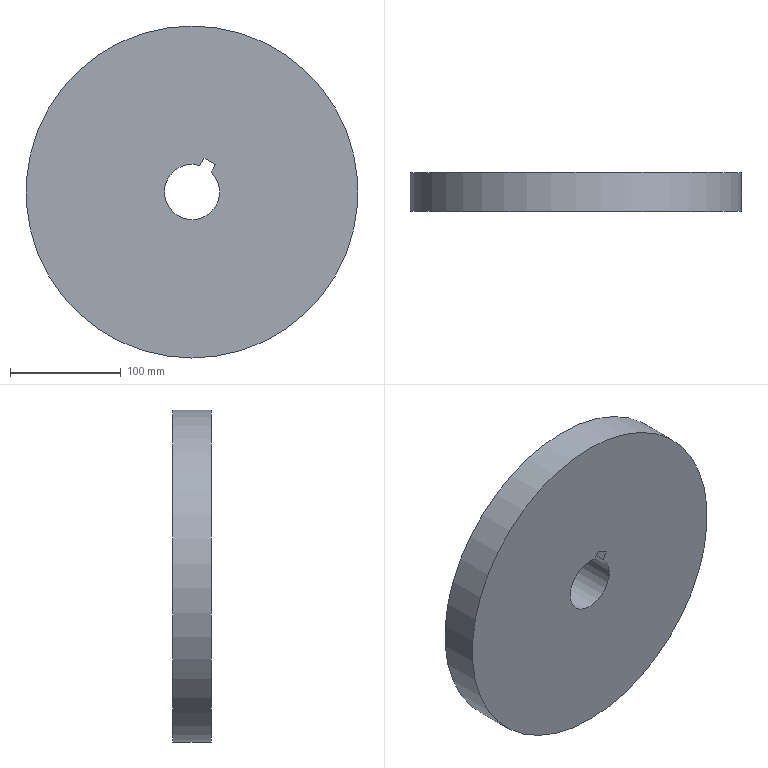Component | NX | TAS | 1 solid | 7 faces | box 300 x 35 x 300 mm | volume 2402240 mm3 | plane 5 | cylinder 2 | commonest cylinder face diameters 300 x1 50 x1
STEP:
#1=CARTESIAN_POINT('',(0.,0.,0.));
#2=DIRECTION('',(0.,0.,1.));
#3=DIRECTION('',(1.,0.,0.));
#4=AXIS2_PLACEMENT_3D('',#1,#2,#3);
#5=CARTESIAN_POINT('',(-1145.062,827.425,250.713));
#6=VERTEX_POINT('',#5);
#7=CARTESIAN_POINT('',(-1148.928,827.425,244.018));
#8=VERTEX_POINT('',#7);
#9=CARTESIAN_POINT('',(-1145.062,827.425,250.713));
#10=DIRECTION('',(-0.5,0.,-0.866));
#11=VECTOR('',#10,1.);
#12=LINE('',#9,#11);
#13=CARTESIAN_POINT('',(-1145.062,792.425,250.713));
#14=DIRECTION('',(0.866,0.,-0.5));
#15=DIRECTION('',(0.5,0.,0.866));
#16=AXIS2_PLACEMENT_3D('',#13,#14,#15);
#17=PLANE('',#16);
#18=CARTESIAN_POINT('',(0.,-35.));
#19=DIRECTION('',(-1.,0.));
#20=VECTOR('',#19,1.);
#21=LINE('',#18,#20);
#22=(GEOMETRIC_REPRESENTATION_CONTEXT(2)PARAMETRIC_REPRESENTATION_CONTEXT()REPRESENTATION_CONTEXT('',''));
#23=DEFINITIONAL_REPRESENTATION('',(#21),#22);
#24=PCURVE('',#17,#23);
#25=CARTESIAN_POINT('',(-1155.866,827.425,220.));
#26=DIRECTION('',(0.,-1.,0.));
#27=DIRECTION('',(-0.5,0.,-0.866));
#28=AXIS2_PLACEMENT_3D('',#25,#26,#27);
#29=PLANE('',#28);
#30=CARTESIAN_POINT('',(-32.,-6.));
#31=DIRECTION('',(1.,-0.));
#32=VECTOR('',#31,1.);
#33=LINE('',#30,#32);
#34=(GEOMETRIC_REPRESENTATION_CONTEXT(2)PARAMETRIC_REPRESENTATION_CONTEXT()REPRESENTATION_CONTEXT('',''));
#35=DEFINITIONAL_REPRESENTATION('',(#33),#34);
#36=PCURVE('',#29,#35);
#37=SURFACE_CURVE('',#12,(#24,#36),.PCURVE_S1.);
#38=EDGE_CURVE('',#6,#8,#37,.T.);
#39=ORIENTED_EDGE('',*,*,#38,.F.);
#40=CARTESIAN_POINT('',(-1145.062,792.425,250.713));
#41=VERTEX_POINT('',#40);
#42=CARTESIAN_POINT('',(-1145.062,792.425,250.713));
#43=DIRECTION('',(0.,1.,0.));
#44=VECTOR('',#43,1.);
#45=LINE('',#42,#44);
#46=CARTESIAN_POINT('',(0.,0.));
#47=DIRECTION('',(0.,-1.));
#48=VECTOR('',#47,1.);
#49=LINE('',#46,#48);
#50=(GEOMETRIC_REPRESENTATION_CONTEXT(2)PARAMETRIC_REPRESENTATION_CONTEXT()REPRESENTATION_CONTEXT('',''));
#51=DEFINITIONAL_REPRESENTATION('',(#49),#50);
#52=PCURVE('',#17,#51);
#53=CARTESIAN_POINT('',(-1134.67,792.425,244.713));
#54=DIRECTION('',(-0.5,0.,-0.866));
#55=DIRECTION('',(0.866,0.,-0.5));
#56=AXIS2_PLACEMENT_3D('',#53,#54,#55);
#57=PLANE('',#56);
#58=CARTESIAN_POINT('',(-12.,0.));
#59=DIRECTION('',(0.,-1.));
#60=VECTOR('',#59,1.);
#61=LINE('',#58,#60);
#62=(GEOMETRIC_REPRESENTATION_CONTEXT(2)PARAMETRIC_REPRESENTATION_CONTEXT()REPRESENTATION_CONTEXT('',''));
#63=DEFINITIONAL_REPRESENTATION('',(#61),#62);
#64=PCURVE('',#57,#63);
#65=SURFACE_CURVE('',#45,(#52,#64),.PCURVE_S1.);
#66=EDGE_CURVE('',#41,#6,#65,.T.);
#67=ORIENTED_EDGE('',*,*,#66,.F.);
#68=CARTESIAN_POINT('',(-1148.928,792.425,244.018));
#69=VERTEX_POINT('',#68);
#70=CARTESIAN_POINT('',(-1145.062,792.425,250.713));
#71=DIRECTION('',(-0.5,0.,-0.866));
#72=VECTOR('',#71,1.);
#73=LINE('',#70,#72);
#74=CARTESIAN_POINT('',(0.,0.));
#75=DIRECTION('',(-1.,0.));
#76=VECTOR('',#75,1.);
#77=LINE('',#74,#76);
#78=(GEOMETRIC_REPRESENTATION_CONTEXT(2)PARAMETRIC_REPRESENTATION_CONTEXT()REPRESENTATION_CONTEXT('',''));
#79=DEFINITIONAL_REPRESENTATION('',(#77),#78);
#80=PCURVE('',#17,#79);
#81=CARTESIAN_POINT('',(-1155.866,792.425,220.));
#82=DIRECTION('',(0.,-1.,0.));
#83=DIRECTION('',(-0.5,0.,-0.866));
#84=AXIS2_PLACEMENT_3D('',#81,#82,#83);
#85=PLANE('',#84);
#86=CARTESIAN_POINT('',(-32.,-6.));
#87=DIRECTION('',(1.,-0.));
#88=VECTOR('',#87,1.);
#89=LINE('',#86,#88);
#90=(GEOMETRIC_REPRESENTATION_CONTEXT(2)PARAMETRIC_REPRESENTATION_CONTEXT()REPRESENTATION_CONTEXT('',''));
#91=DEFINITIONAL_REPRESENTATION('',(#89),#90);
#92=PCURVE('',#85,#91);
#93=SURFACE_CURVE('',#73,(#80,#92),.PCURVE_S1.);
#94=EDGE_CURVE('',#41,#69,#93,.T.);
#95=ORIENTED_EDGE('',*,*,#94,.T.);
#96=CARTESIAN_POINT('',(-1148.928,792.425,244.018));
#97=DIRECTION('',(0.,1.,0.));
#98=VECTOR('',#97,1.);
#99=LINE('',#96,#98);
#100=CARTESIAN_POINT('',(-7.731,0.));
#101=DIRECTION('',(0.,-1.));
#102=VECTOR('',#101,1.);
#103=LINE('',#100,#102);
#104=(GEOMETRIC_REPRESENTATION_CONTEXT(2)PARAMETRIC_REPRESENTATION_CONTEXT()REPRESENTATION_CONTEXT('',''));
#105=DEFINITIONAL_REPRESENTATION('',(#103),#104);
#106=PCURVE('',#17,#105);
#107=CARTESIAN_POINT('',(-1155.866,792.425,220.));
#108=DIRECTION('',(0.,1.,0.));
#109=DIRECTION('',(0.5,0.,0.866));
#110=AXIS2_PLACEMENT_3D('',#107,#108,#109);
#111=CYLINDRICAL_SURFACE('',#110,25.);
#112=CARTESIAN_POINT('',(6.041,0.));
#113=DIRECTION('',(0.,1.));
#114=VECTOR('',#113,1.);
#115=LINE('',#112,#114);
#116=(GEOMETRIC_REPRESENTATION_CONTEXT(2)PARAMETRIC_REPRESENTATION_CONTEXT()REPRESENTATION_CONTEXT('',''));
#117=DEFINITIONAL_REPRESENTATION('',(#115),#116);
#118=PCURVE('',#111,#117);
#119=SURFACE_CURVE('',#99,(#106,#118),.PCURVE_S1.);
#120=EDGE_CURVE('',#69,#8,#119,.T.);
#121=ORIENTED_EDGE('',*,*,#120,.T.);
#122=EDGE_LOOP('',(#39,#67,#95,#121));
#123=FACE_BOUND('',#122,.T.);
#124=ADVANCED_FACE('',(#123),#17,.T.);
#125=CARTESIAN_POINT('',(-1134.67,827.425,244.713));
#126=VERTEX_POINT('',#125);
#127=CARTESIAN_POINT('',(-1134.67,827.425,244.713));
#128=DIRECTION('',(-0.866,0.,0.5));
#129=VECTOR('',#128,1.);
#130=LINE('',#127,#129);
#131=CARTESIAN_POINT('',(0.,-35.));
#132=DIRECTION('',(-1.,0.));
#133=VECTOR('',#132,1.);
#134=LINE('',#131,#133);
#135=(GEOMETRIC_REPRESENTATION_CONTEXT(2)PARAMETRIC_REPRESENTATION_CONTEXT()REPRESENTATION_CONTEXT('',''));
#136=DEFINITIONAL_REPRESENTATION('',(#134),#135);
#137=PCURVE('',#57,#136);
#138=CARTESIAN_POINT('',(-32.,6.));
#139=DIRECTION('',(-0.,-1.));
#140=VECTOR('',#139,1.);
#141=LINE('',#138,#140);
#142=(GEOMETRIC_REPRESENTATION_CONTEXT(2)PARAMETRIC_REPRESENTATION_CONTEXT()REPRESENTATION_CONTEXT('',''));
#143=DEFINITIONAL_REPRESENTATION('',(#141),#142);
#144=PCURVE('',#29,#143);
#145=SURFACE_CURVE('',#130,(#137,#144),.PCURVE_S1.);
#146=EDGE_CURVE('',#126,#6,#145,.T.);
#147=ORIENTED_EDGE('',*,*,#146,.F.);
#148=CARTESIAN_POINT('',(-1134.67,792.425,244.713));
#149=VERTEX_POINT('',#148);
#150=CARTESIAN_POINT('',(-1134.67,792.425,244.713));
#151=DIRECTION('',(0.,1.,0.));
#152=VECTOR('',#151,1.);
#153=LINE('',#150,#152);
#154=CARTESIAN_POINT('',(0.,0.));
#155=DIRECTION('',(0.,-1.));
#156=VECTOR('',#155,1.);
#157=LINE('',#154,#156);
#158=(GEOMETRIC_REPRESENTATION_CONTEXT(2)PARAMETRIC_REPRESENTATION_CONTEXT()REPRESENTATION_CONTEXT('',''));
#159=DEFINITIONAL_REPRESENTATION('',(#157),#158);
#160=PCURVE('',#57,#159);
#161=CARTESIAN_POINT('',(-1138.535,792.425,238.018));
#162=DIRECTION('',(-0.866,0.,0.5));
#163=DIRECTION('',(-0.5,0.,-0.866));
#164=AXIS2_PLACEMENT_3D('',#161,#162,#163);
#165=PLANE('',#164);
#166=CARTESIAN_POINT('',(-7.731,0.));
#167=DIRECTION('',(0.,-1.));
#168=VECTOR('',#167,1.);
#169=LINE('',#166,#168);
#170=(GEOMETRIC_REPRESENTATION_CONTEXT(2)PARAMETRIC_REPRESENTATION_CONTEXT()REPRESENTATION_CONTEXT('',''));
#171=DEFINITIONAL_REPRESENTATION('',(#169),#170);
#172=PCURVE('',#165,#171);
#173=SURFACE_CURVE('',#153,(#160,#172),.PCURVE_S1.);
#174=EDGE_CURVE('',#149,#126,#173,.T.);
#175=ORIENTED_EDGE('',*,*,#174,.F.);
#176=CARTESIAN_POINT('',(-1134.67,792.425,244.713));
#177=DIRECTION('',(-0.866,0.,0.5));
#178=VECTOR('',#177,1.);
#179=LINE('',#176,#178);
#180=CARTESIAN_POINT('',(0.,0.));
#181=DIRECTION('',(-1.,0.));
#182=VECTOR('',#181,1.);
#183=LINE('',#180,#182);
#184=(GEOMETRIC_REPRESENTATION_CONTEXT(2)PARAMETRIC_REPRESENTATION_CONTEXT()REPRESENTATION_CONTEXT('',''));
#185=DEFINITIONAL_REPRESENTATION('',(#183),#184);
#186=PCURVE('',#57,#185);
#187=CARTESIAN_POINT('',(-32.,6.));
#188=DIRECTION('',(-0.,-1.));
#189=VECTOR('',#188,1.);
#190=LINE('',#187,#189);
#191=(GEOMETRIC_REPRESENTATION_CONTEXT(2)PARAMETRIC_REPRESENTATION_CONTEXT()REPRESENTATION_CONTEXT('',''));
#192=DEFINITIONAL_REPRESENTATION('',(#190),#191);
#193=PCURVE('',#85,#192);
#194=SURFACE_CURVE('',#179,(#186,#193),.PCURVE_S1.);
#195=EDGE_CURVE('',#149,#41,#194,.T.);
#196=ORIENTED_EDGE('',*,*,#195,.T.);
#197=ORIENTED_EDGE('',*,*,#66,.T.);
#198=EDGE_LOOP('',(#147,#175,#196,#197));
#199=FACE_BOUND('',#198,.T.);
#200=ADVANCED_FACE('',(#199),#57,.T.);
#201=CARTESIAN_POINT('',(-1138.535,827.425,238.018));
#202=VERTEX_POINT('',#201);
#203=CARTESIAN_POINT('',(-1138.535,827.425,238.018));
#204=DIRECTION('',(0.5,0.,0.866));
#205=VECTOR('',#204,1.);
#206=LINE('',#203,#205);
#207=CARTESIAN_POINT('',(0.,-35.));
#208=DIRECTION('',(-1.,0.));
#209=VECTOR('',#208,1.);
#210=LINE('',#207,#209);
#211=(GEOMETRIC_REPRESENTATION_CONTEXT(2)PARAMETRIC_REPRESENTATION_CONTEXT()REPRESENTATION_CONTEXT('',''));
#212=DEFINITIONAL_REPRESENTATION('',(#210),#211);
#213=PCURVE('',#165,#212);
#214=CARTESIAN_POINT('',(-24.269,6.));
#215=DIRECTION('',(-1.,-0.));
#216=VECTOR('',#215,1.);
#217=LINE('',#214,#216);
#218=(GEOMETRIC_REPRESENTATION_CONTEXT(2)PARAMETRIC_REPRESENTATION_CONTEXT()REPRESENTATION_CONTEXT('',''));
#219=DEFINITIONAL_REPRESENTATION('',(#217),#218);
#220=PCURVE('',#29,#219);
#221=SURFACE_CURVE('',#206,(#213,#220),.PCURVE_S1.);
#222=EDGE_CURVE('',#202,#126,#221,.T.);
#223=ORIENTED_EDGE('',*,*,#222,.F.);
#224=CARTESIAN_POINT('',(-1138.535,792.425,238.018));
#225=VERTEX_POINT('',#224);
#226=CARTESIAN_POINT('',(-1138.535,792.425,238.018));
#227=DIRECTION('',(0.,1.,0.));
#228=VECTOR('',#227,1.);
#229=LINE('',#226,#228);
#230=CARTESIAN_POINT('',(0.,0.));
#231=DIRECTION('',(0.,-1.));
#232=VECTOR('',#231,1.);
#233=LINE('',#230,#232);
#234=(GEOMETRIC_REPRESENTATION_CONTEXT(2)PARAMETRIC_REPRESENTATION_CONTEXT()REPRESENTATION_CONTEXT('',''));
#235=DEFINITIONAL_REPRESENTATION('',(#233),#234);
#236=PCURVE('',#165,#235);
#237=CARTESIAN_POINT('',(0.2424,0.));
#238=DIRECTION('',(0.,1.));
#239=VECTOR('',#238,1.);
#240=LINE('',#237,#239);
#241=(GEOMETRIC_REPRESENTATION_CONTEXT(2)PARAMETRIC_REPRESENTATION_CONTEXT()REPRESENTATION_CONTEXT('',''));
#242=DEFINITIONAL_REPRESENTATION('',(#240),#241);
#243=PCURVE('',#111,#242);
#244=SURFACE_CURVE('',#229,(#236,#243),.PCURVE_S1.);
#245=EDGE_CURVE('',#225,#202,#244,.T.);
#246=ORIENTED_EDGE('',*,*,#245,.F.);
#247=CARTESIAN_POINT('',(-1138.535,792.425,238.018));
#248=DIRECTION('',(0.5,0.,0.866));
#249=VECTOR('',#248,1.);
#250=LINE('',#247,#249);
#251=CARTESIAN_POINT('',(0.,0.));
#252=DIRECTION('',(-1.,0.));
#253=VECTOR('',#252,1.);
#254=LINE('',#251,#253);
#255=(GEOMETRIC_REPRESENTATION_CONTEXT(2)PARAMETRIC_REPRESENTATION_CONTEXT()REPRESENTATION_CONTEXT('',''));
#256=DEFINITIONAL_REPRESENTATION('',(#254),#255);
#257=PCURVE('',#165,#256);
#258=CARTESIAN_POINT('',(-24.269,6.));
#259=DIRECTION('',(-1.,-0.));
#260=VECTOR('',#259,1.);
#261=LINE('',#258,#260);
#262=(GEOMETRIC_REPRESENTATION_CONTEXT(2)PARAMETRIC_REPRESENTATION_CONTEXT()REPRESENTATION_CONTEXT('',''));
#263=DEFINITIONAL_REPRESENTATION('',(#261),#262);
#264=PCURVE('',#85,#263);
#265=SURFACE_CURVE('',#250,(#257,#264),.PCURVE_S1.);
#266=EDGE_CURVE('',#225,#149,#265,.T.);
#267=ORIENTED_EDGE('',*,*,#266,.T.);
#268=ORIENTED_EDGE('',*,*,#174,.T.);
#269=EDGE_LOOP('',(#223,#246,#267,#268));
#270=FACE_BOUND('',#269,.T.);
#271=ADVANCED_FACE('',(#270),#165,.T.);
#272=CARTESIAN_POINT('',(-1025.962,792.425,145.));
#273=VERTEX_POINT('',#272);
#274=CARTESIAN_POINT('',(-1155.866,792.425,220.));
#275=DIRECTION('',(0.,-1.,0.));
#276=DIRECTION('',(0.866,0.,-0.5));
#277=AXIS2_PLACEMENT_3D('',#274,#275,#276);
#278=CIRCLE('',#277,150.);
#279=CARTESIAN_POINT('',(-1155.866,792.425,220.));
#280=DIRECTION('',(0.,1.,0.));
#281=DIRECTION('',(0.5,0.,0.866));
#282=AXIS2_PLACEMENT_3D('',#279,#280,#281);
#283=CYLINDRICAL_SURFACE('',#282,150.);
#284=CARTESIAN_POINT('',(7.854,0.));
#285=DIRECTION('',(-1.,0.));
#286=VECTOR('',#285,1.);
#287=LINE('',#284,#286);
#288=(GEOMETRIC_REPRESENTATION_CONTEXT(2)PARAMETRIC_REPRESENTATION_CONTEXT()REPRESENTATION_CONTEXT('',''));
#289=DEFINITIONAL_REPRESENTATION('',(#287),#288);
#290=PCURVE('',#283,#289);
#291=CARTESIAN_POINT('',(0.,0.));
#292=DIRECTION('',(0.,1.));
#293=AXIS2_PLACEMENT_2D('',#291,#292);
#294=CIRCLE('',#293,150.);
#295=(GEOMETRIC_REPRESENTATION_CONTEXT(2)PARAMETRIC_REPRESENTATION_CONTEXT()REPRESENTATION_CONTEXT('',''));
#296=DEFINITIONAL_REPRESENTATION('',(#294),#295);
#297=PCURVE('',#85,#296);
#298=SURFACE_CURVE('',#278,(#290,#297),.PCURVE_S1.);
#299=EDGE_CURVE('',#273,#273,#298,.T.);
#300=ORIENTED_EDGE('',*,*,#299,.F.);
#301=CARTESIAN_POINT('',(-1025.962,827.425,145.));
#302=VERTEX_POINT('',#301);
#303=CARTESIAN_POINT('',(-1025.962,792.425,145.));
#304=CARTESIAN_POINT('',(-1025.962,827.425,145.));
#305=B_SPLINE_CURVE_WITH_KNOTS('',1,(#303,#304),.UNSPECIFIED.,.F.,.F.,(2,2),(0.,35.),.PIECEWISE_BEZIER_KNOTS.);
#306=CARTESIAN_POINT('',(7.854,0.));
#307=DIRECTION('',(0.,1.));
#308=VECTOR('',#307,1.);
#309=LINE('',#306,#308);
#310=(GEOMETRIC_REPRESENTATION_CONTEXT(2)PARAMETRIC_REPRESENTATION_CONTEXT()REPRESENTATION_CONTEXT('',''));
#311=DEFINITIONAL_REPRESENTATION('',(#309),#310);
#312=PCURVE('',#283,#311);
#313=CARTESIAN_POINT('',(1.571,0.));
#314=DIRECTION('',(0.,1.));
#315=VECTOR('',#314,1.);
#316=LINE('',#313,#315);
#317=(GEOMETRIC_REPRESENTATION_CONTEXT(2)PARAMETRIC_REPRESENTATION_CONTEXT()REPRESENTATION_CONTEXT('',''));
#318=DEFINITIONAL_REPRESENTATION('',(#316),#317);
#319=PCURVE('',#283,#318);
#320=SEAM_CURVE('',#305,(#312,#319),.PCURVE_S1.);
#321=EDGE_CURVE('',#273,#302,#320,.T.);
#322=ORIENTED_EDGE('',*,*,#321,.T.);
#323=CARTESIAN_POINT('',(-1155.866,827.425,220.));
#324=DIRECTION('',(0.,-1.,0.));
#325=DIRECTION('',(0.866,0.,-0.5));
#326=AXIS2_PLACEMENT_3D('',#323,#324,#325);
#327=CIRCLE('',#326,150.);
#328=CARTESIAN_POINT('',(7.854,35.));
#329=DIRECTION('',(-1.,0.));
#330=VECTOR('',#329,1.);
#331=LINE('',#328,#330);
#332=(GEOMETRIC_REPRESENTATION_CONTEXT(2)PARAMETRIC_REPRESENTATION_CONTEXT()REPRESENTATION_CONTEXT('',''));
#333=DEFINITIONAL_REPRESENTATION('',(#331),#332);
#334=PCURVE('',#283,#333);
#335=CARTESIAN_POINT('',(0.,0.));
#336=DIRECTION('',(0.,1.));
#337=AXIS2_PLACEMENT_2D('',#335,#336);
#338=CIRCLE('',#337,150.);
#339=(GEOMETRIC_REPRESENTATION_CONTEXT(2)PARAMETRIC_REPRESENTATION_CONTEXT()REPRESENTATION_CONTEXT('',''));
#340=DEFINITIONAL_REPRESENTATION('',(#338),#339);
#341=PCURVE('',#29,#340);
#342=SURFACE_CURVE('',#327,(#334,#341),.PCURVE_S1.);
#343=EDGE_CURVE('',#302,#302,#342,.T.);
#344=ORIENTED_EDGE('',*,*,#343,.T.);
#345=ORIENTED_EDGE('',*,*,#321,.F.);
#346=EDGE_LOOP('',(#300,#322,#344,#345));
#347=FACE_BOUND('',#346,.T.);
#348=ADVANCED_FACE('',(#347),#283,.T.);
#349=ORIENTED_EDGE('',*,*,#245,.F.);
#350=CARTESIAN_POINT('',(-1155.866,792.425,220.));
#351=DIRECTION('',(0.,-1.,0.));
#352=DIRECTION('',(0.866,0.,-0.5));
#353=AXIS2_PLACEMENT_3D('',#350,#351,#352);
#354=CIRCLE('',#353,25.);
#355=CARTESIAN_POINT('',(7.854,0.));
#356=DIRECTION('',(-1.,0.));
#357=VECTOR('',#356,1.);
#358=LINE('',#355,#357);
#359=(GEOMETRIC_REPRESENTATION_CONTEXT(2)PARAMETRIC_REPRESENTATION_CONTEXT()REPRESENTATION_CONTEXT('',''));
#360=DEFINITIONAL_REPRESENTATION('',(#358),#359);
#361=PCURVE('',#111,#360);
#362=CARTESIAN_POINT('',(0.,0.));
#363=DIRECTION('',(-0.,1.));
#364=AXIS2_PLACEMENT_2D('',#362,#363);
#365=CIRCLE('',#364,25.);
#366=(GEOMETRIC_REPRESENTATION_CONTEXT(2)PARAMETRIC_REPRESENTATION_CONTEXT()REPRESENTATION_CONTEXT('',''));
#367=DEFINITIONAL_REPRESENTATION('',(#365),#366);
#368=PCURVE('',#85,#367);
#369=SURFACE_CURVE('',#354,(#361,#368),.PCURVE_S1.);
#370=EDGE_CURVE('',#69,#225,#369,.T.);
#371=ORIENTED_EDGE('',*,*,#370,.F.);
#372=ORIENTED_EDGE('',*,*,#120,.T.);
#373=CARTESIAN_POINT('',(-1155.866,827.425,220.));
#374=DIRECTION('',(0.,-1.,0.));
#375=DIRECTION('',(0.866,0.,-0.5));
#376=AXIS2_PLACEMENT_3D('',#373,#374,#375);
#377=CIRCLE('',#376,25.);
#378=CARTESIAN_POINT('',(7.854,35.));
#379=DIRECTION('',(-1.,0.));
#380=VECTOR('',#379,1.);
#381=LINE('',#378,#380);
#382=(GEOMETRIC_REPRESENTATION_CONTEXT(2)PARAMETRIC_REPRESENTATION_CONTEXT()REPRESENTATION_CONTEXT('',''));
#383=DEFINITIONAL_REPRESENTATION('',(#381),#382);
#384=PCURVE('',#111,#383);
#385=CARTESIAN_POINT('',(0.,0.));
#386=DIRECTION('',(-0.,1.));
#387=AXIS2_PLACEMENT_2D('',#385,#386);
#388=CIRCLE('',#387,25.);
#389=(GEOMETRIC_REPRESENTATION_CONTEXT(2)PARAMETRIC_REPRESENTATION_CONTEXT()REPRESENTATION_CONTEXT('',''));
#390=DEFINITIONAL_REPRESENTATION('',(#388),#389);
#391=PCURVE('',#29,#390);
#392=SURFACE_CURVE('',#377,(#384,#391),.PCURVE_S1.);
#393=EDGE_CURVE('',#8,#202,#392,.T.);
#394=ORIENTED_EDGE('',*,*,#393,.T.);
#395=EDGE_LOOP('',(#349,#371,#372,#394));
#396=FACE_BOUND('',#395,.F.);
#397=ADVANCED_FACE('',(#396),#111,.F.);
#398=ORIENTED_EDGE('',*,*,#299,.T.);
#399=EDGE_LOOP('',(#398));
#400=FACE_BOUND('',#399,.T.);
#401=ORIENTED_EDGE('',*,*,#94,.F.);
#402=ORIENTED_EDGE('',*,*,#195,.F.);
#403=ORIENTED_EDGE('',*,*,#266,.F.);
#404=ORIENTED_EDGE('',*,*,#370,.F.);
#405=EDGE_LOOP('',(#401,#402,#403,#404));
#406=FACE_BOUND('',#405,.T.);
#407=ADVANCED_FACE('',(#400,#406),#85,.T.);
#408=ORIENTED_EDGE('',*,*,#343,.F.);
#409=EDGE_LOOP('',(#408));
#410=FACE_BOUND('',#409,.T.);
#411=ORIENTED_EDGE('',*,*,#38,.T.);
#412=ORIENTED_EDGE('',*,*,#393,.T.);
#413=ORIENTED_EDGE('',*,*,#222,.T.);
#414=ORIENTED_EDGE('',*,*,#146,.T.);
#415=EDGE_LOOP('',(#411,#412,#413,#414));
#416=FACE_BOUND('',#415,.T.);
#417=ADVANCED_FACE('',(#410,#416),#29,.F.);
#418=CLOSED_SHELL('',(#124,#200,#271,#348,#397,#407,#417));
#419=MANIFOLD_SOLID_BREP('',#418);
#420=(LENGTH_UNIT()NAMED_UNIT(*)SI_UNIT(.MILLI.,.METRE.));
#421=UNCERTAINTY_MEASURE_WITH_UNIT(LENGTH_MEASURE(0.000002),#420,'','');
#422=(NAMED_UNIT(*)PLANE_ANGLE_UNIT()SI_UNIT($,.RADIAN.));
#423=(NAMED_UNIT(*)SI_UNIT($,.STERADIAN.)SOLID_ANGLE_UNIT());
#424=(GEOMETRIC_REPRESENTATION_CONTEXT(3)GLOBAL_UNCERTAINTY_ASSIGNED_CONTEXT((#421))GLOBAL_UNIT_ASSIGNED_CONTEXT((#420,#422,#423))REPRESENTATION_CONTEXT('',''));
#425=ADVANCED_BREP_SHAPE_REPRESENTATION('',(#4,#419),#424);